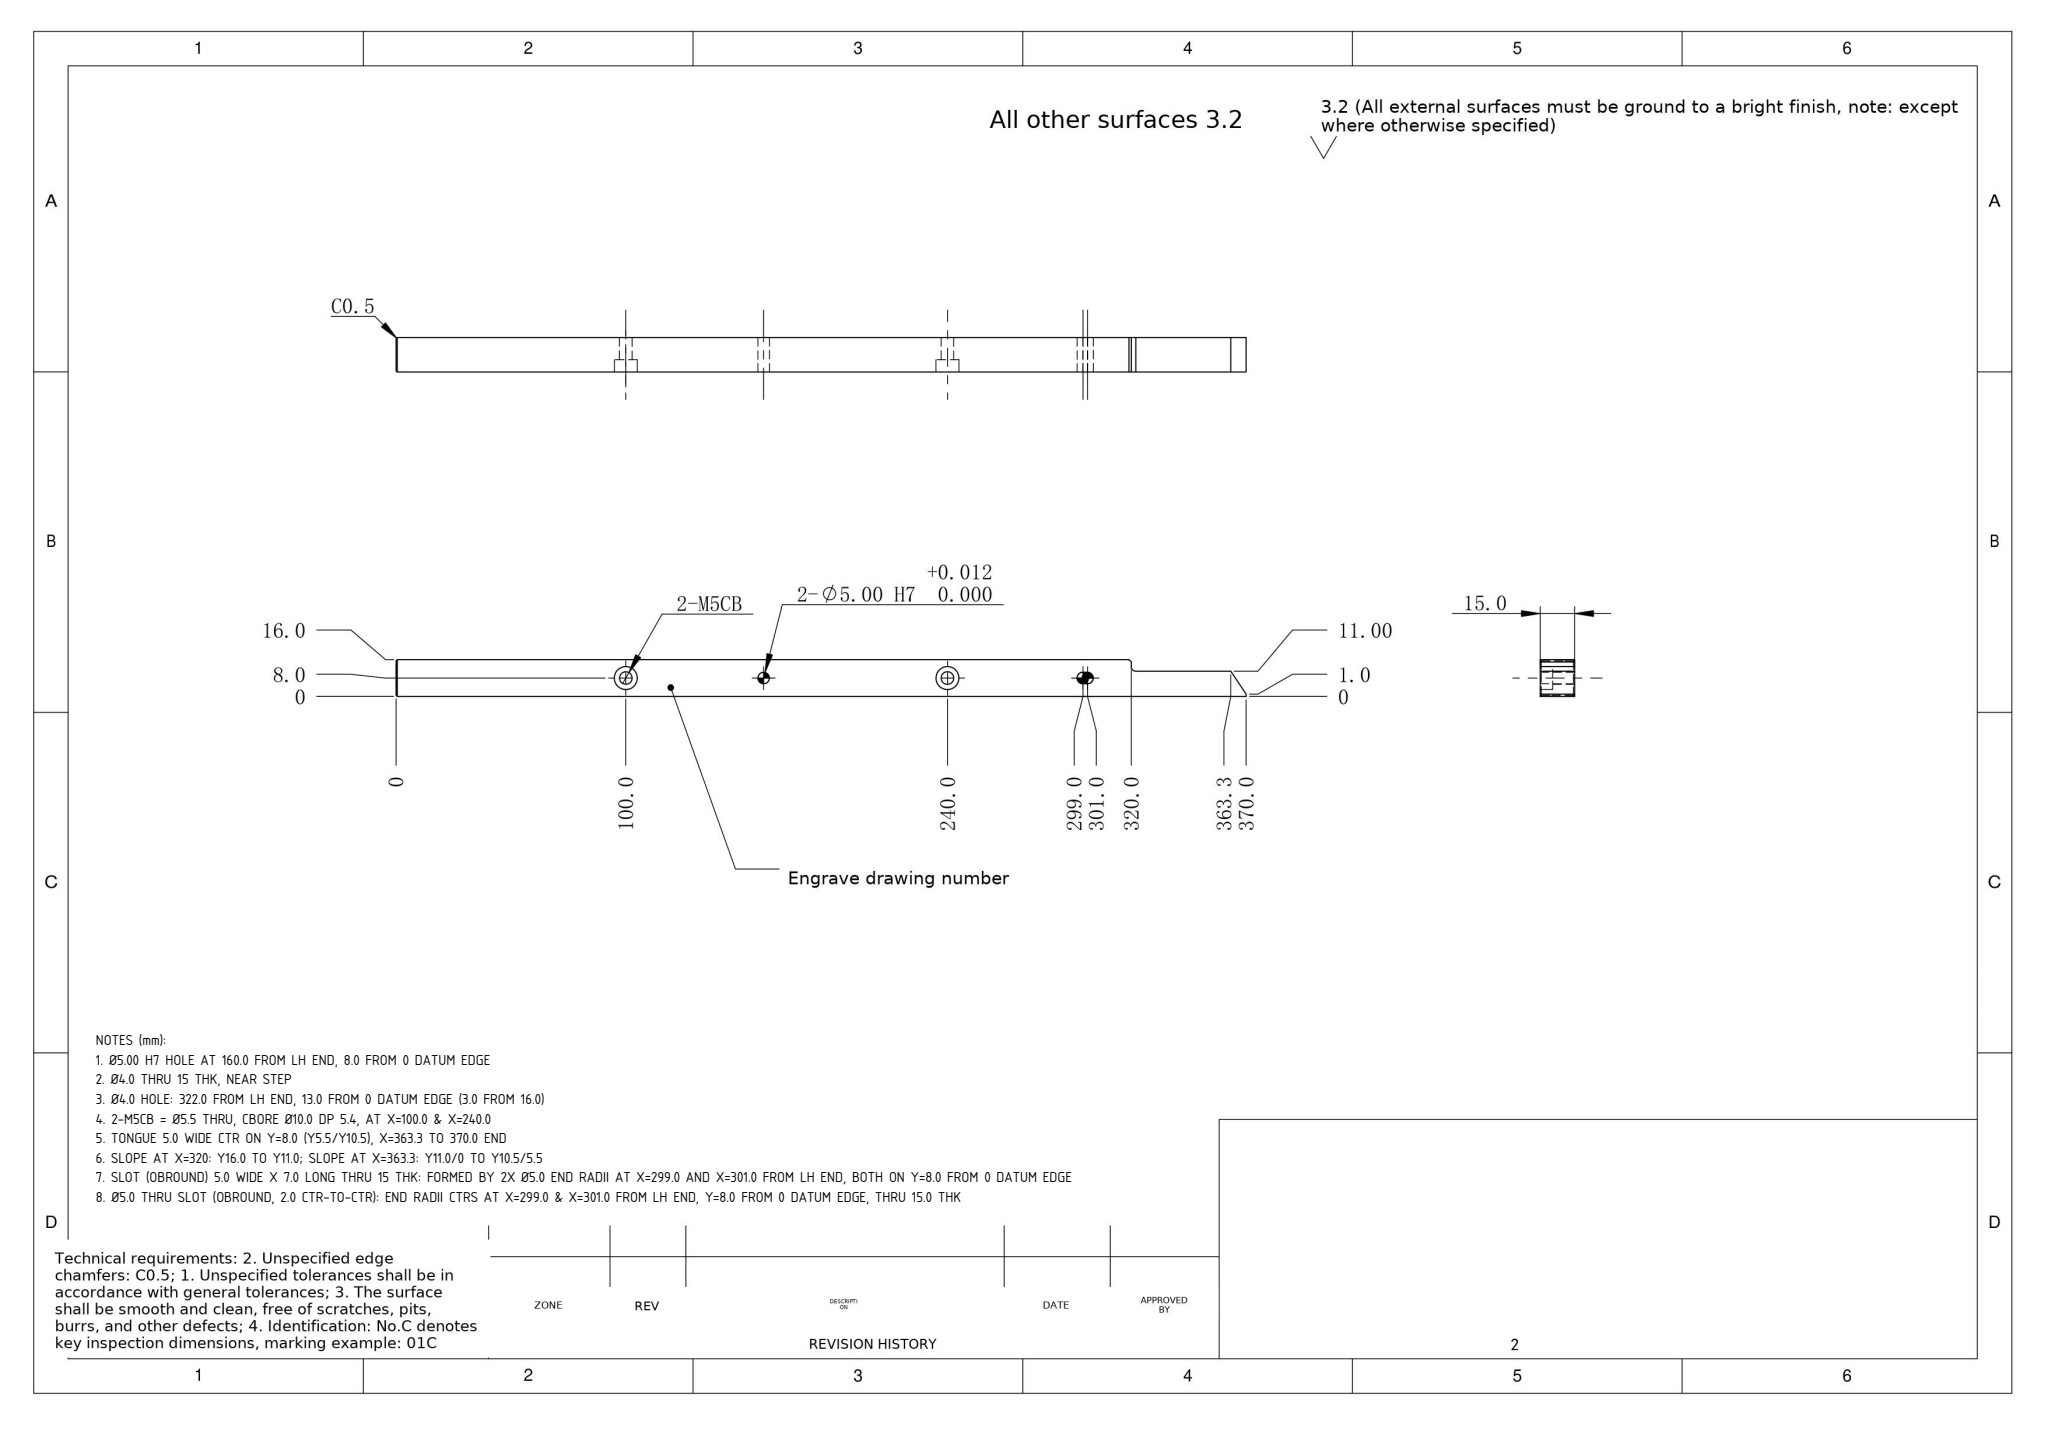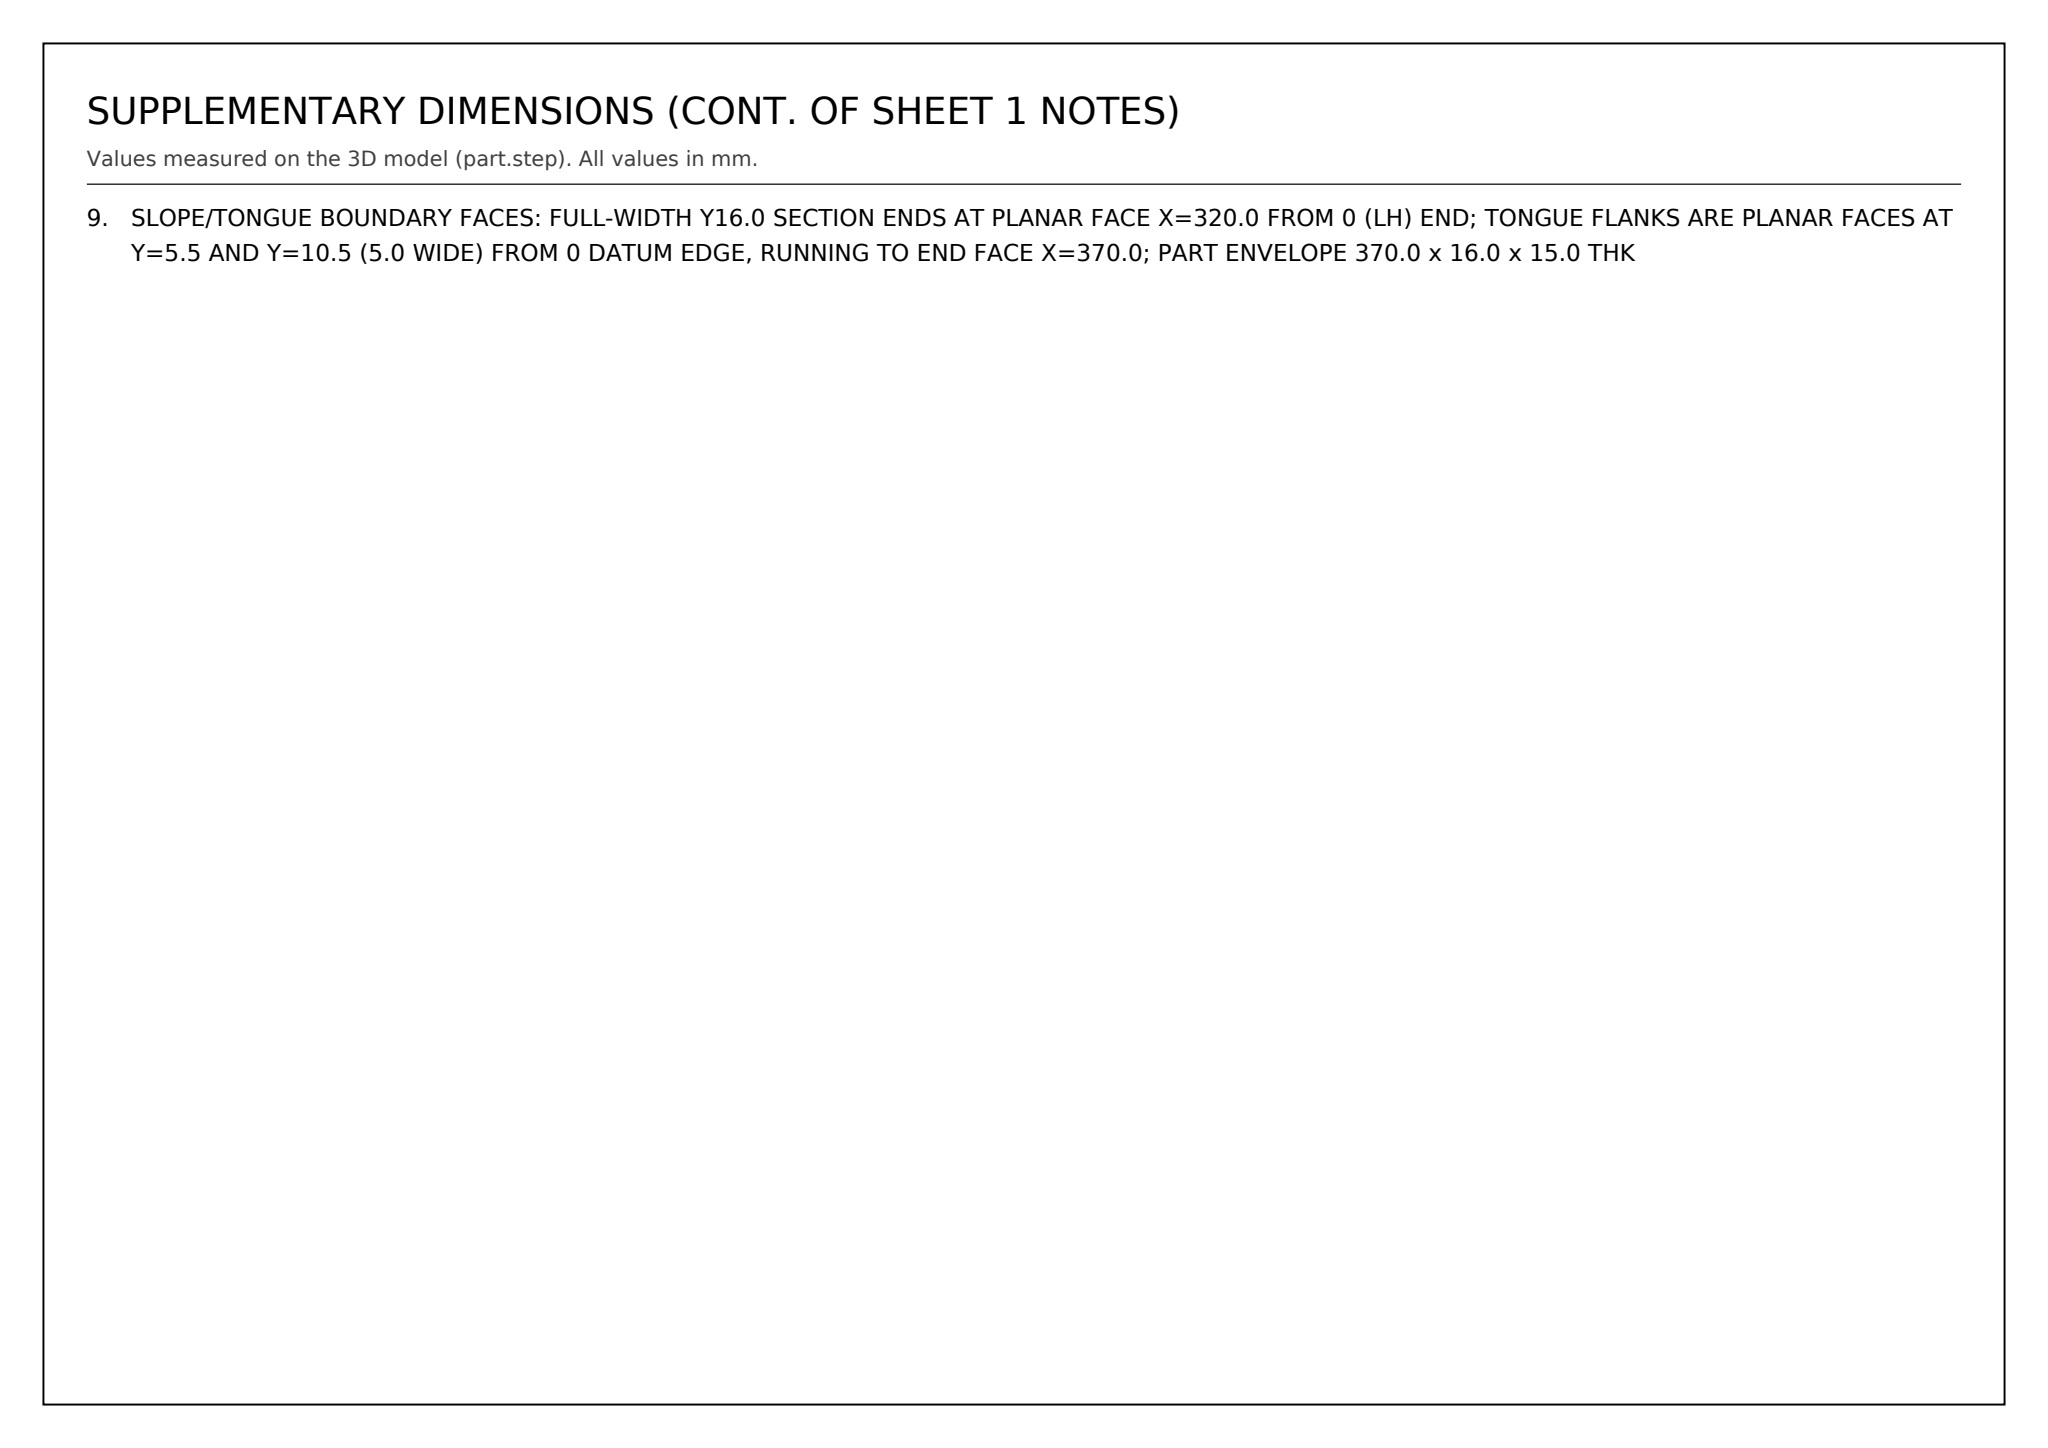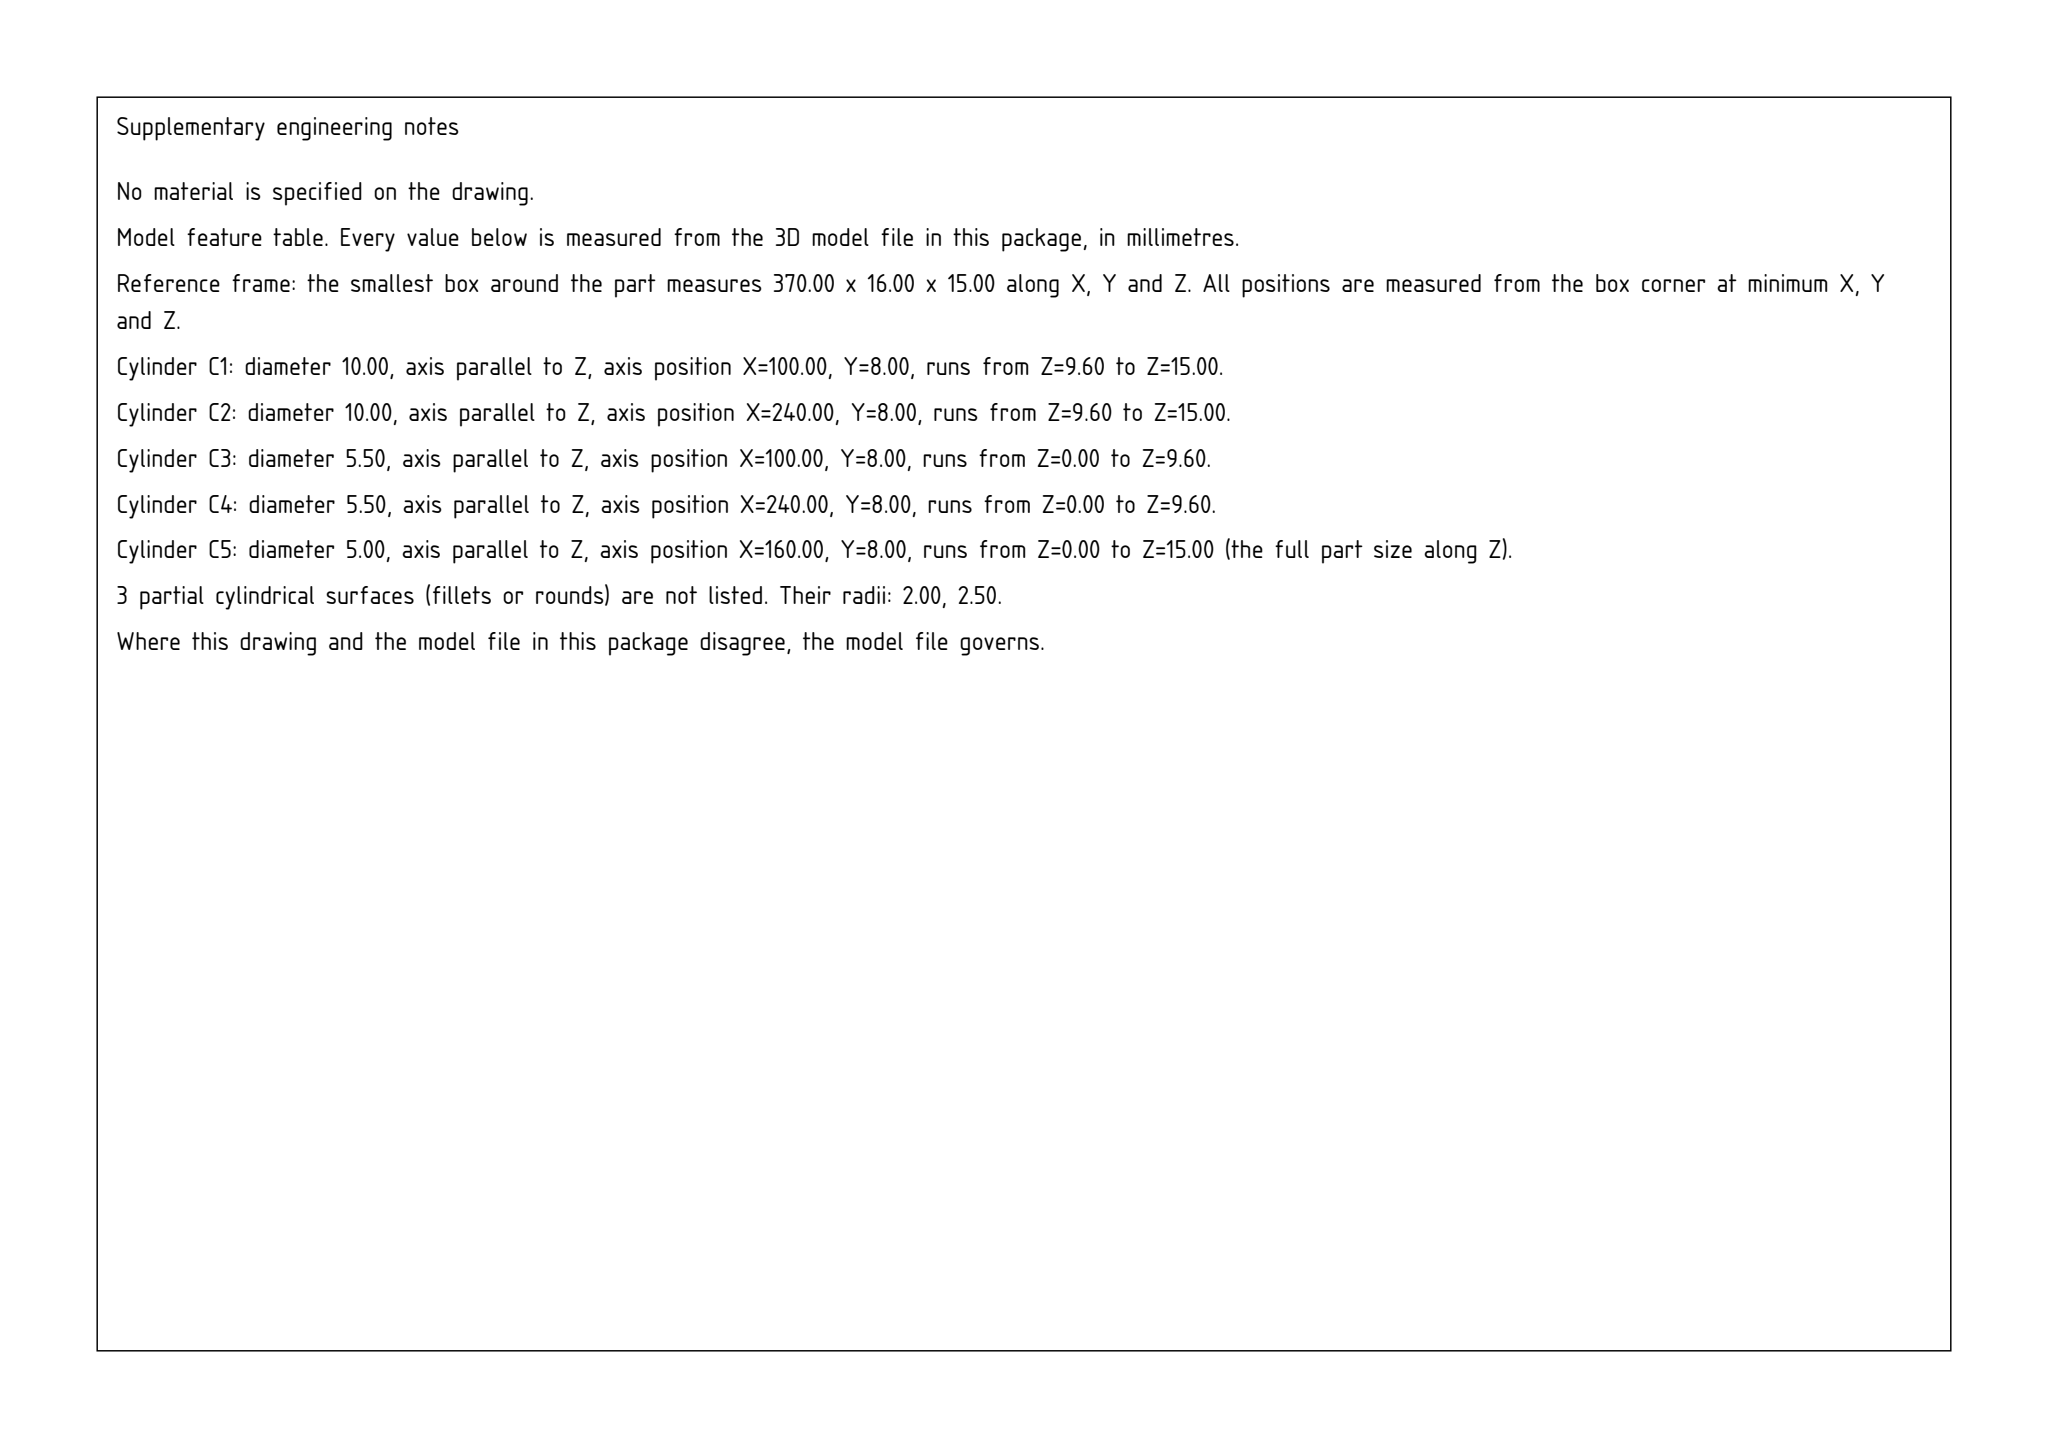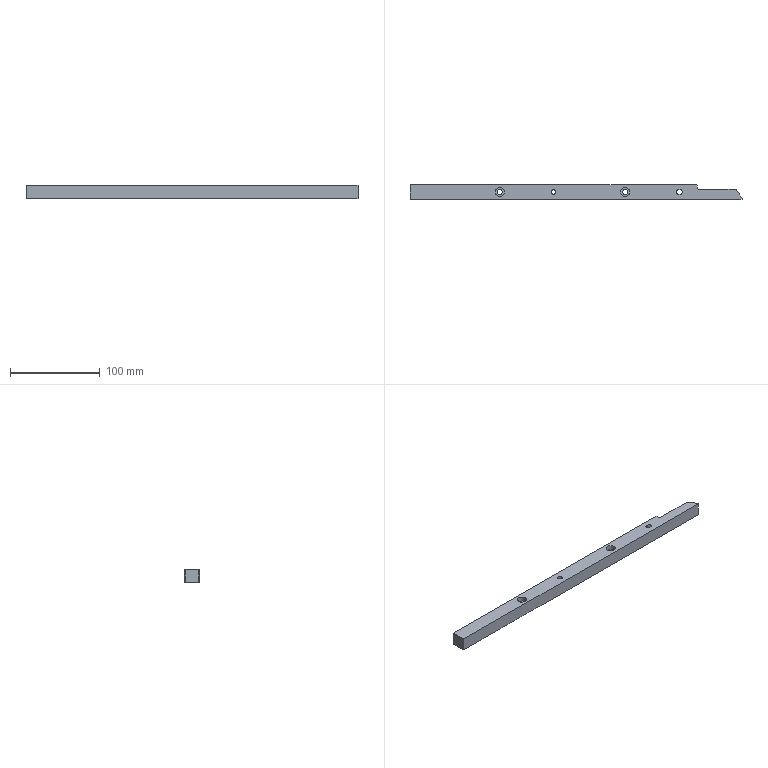Part | SolidWorks | mm | 1 solid | 32 faces | box 370 x 16 x 15 mm | volume 82504 mm3 | plane 18 | cylinder 14 | commonest cylinder face diameters 5 x5 10 x4 5.5 x4 4 x1
Drawing notes:
Ø5.00 H7 HOLE AT 160.0 FROM LH END, 8.0 FROM 0 DATUM EDGE | from the solid: cyl dia 5.0 axis z at (160.0, 8.0), len 15.0 (thru)
Ø4.0 THRU 15 THK, NEAR STEP | from the solid: cyl dia 4.0 axis z at (322.0, 13.0), len 15.0 = part thickness
Ø4.0 HOLE: 322.0 FROM LH END, 13.0 FROM 0 DATUM EDGE (3.0 FROM 16.0) | from the solid: cyl dia 4.0 pos x=322.0, y=13.0; y planes 0.0 and 16.0
2-M5CB = Ø5.5 THRU, CBORE Ø10.0 DP 5.4, AT X=100.0 & X=240.0 | from the solid: cyl Ø5.5 z @ (100,8) & (240,8) L9.6 thru; cyl Ø10.0 z same pos L5.4
TONGUE 5.0 WIDE CTR ON Y=8.0 (Y5.5/Y10.5), X=363.3 TO 370.0 END | from the solid: y-planes at 5.5 and 10.5; x-planes 370.0 end, 363.3 sloped face in view
SLOPE AT X=320: Y16.0 TO Y11.0; SLOPE AT X=363.3: Y11.0/0 TO Y10.5/5.5 | from the solid: y-planes 0,5.5,10.5,11.0,16.0; x-planes 0,320.0,370.0; no cones/fillets
SLOT (OBROUND) 5.0 WIDE X 7.0 LONG THRU 15 THK: FORMED BY 2X Ø5.0 END RADII AT X=299.0 AND X=301.0 FROM LH END, BOTH ON Y=8.0 FROM 0 DATUM EDGE | from the solid: cylinders: [5.0,'z',[299.0,8.0],15.0] and [5.0,'z',[301.0,8.0],15.0]; bbox z = 15.0
Ø5.0 THRU SLOT (OBROUND, 2.0 CTR-TO-CTR): END RADII CTRS AT X=299.0 & X=301.0 FROM LH END, Y=8.0 FROM 0 DATUM EDGE, THRU 15.0 THK | from the solid: cylinders: [5.0,'z',[299.0,8.0],15.0] and [5.0,'z',[301.0,8.0],15.0]; bbox_xyz z=15.0
SLOPE/TONGUE BOUNDARY FACES: FULL-WIDTH Y16.0 SECTION ENDS AT PLANAR FACE X=320.0 FROM 0 (LH) END; TONGUE FLANKS ARE PLANAR FACES AT Y=5.5 AND Y=10.5 (5.0 WIDE) FROM 0 DATUM EDGE, RUNNING TO END FACE X=370.0; PART ENVELOPE 370.0 x 16.0 x 15.0 THK | from the solid: axis_planes[x,0.0], [x,320.0], [x,370.0], [y,5.5], [y,10.5], [y,16.0], [z,0.0], [z,15.0]; bbox_xyz [370.0,16.0,15.0]
build123d program:
from build123d import *

# Parameters (mm, degrees)
SKETCH1_W                                       = 370
SKETCH1_H                                       = 16
BOSS_EXTRUDE1_DEPTH                             = 15
M5_HEX_SOCKET_HEAD_CAP_SCREW_CBORE1_D           = 5.5
M5_HEX_SOCKET_HEAD_CAP_SCREW_CBORE1_CBORE_D     = 10
M5_HEX_SOCKET_HEAD_CAP_SCREW_CBORE1_CBORE_DEPTH = 5.4
LPATTERN1_COUNT                                 = 2
LPATTERN1_PITCH                                 = 140
CHAMFER1_SIZE                                   = 15
CHAMFER1_SIZE2                                  = 10
CHAMFER2_SIZE                                   = 0.5
SKETCH4_R                                       = 2.5
CUT_EXTRUDE1_DEPTH                              = 371.649
SKETCH5_W                                       = 50
SKETCH5_H                                       = 5
CUT_EXTRUDE2_DEPTH                              = 371.649
CHAMFER3_SIZE                                   = 1
FILLET1_R                                       = 2


with BuildPart() as part:
    # Sketch1 → Boss-Extrude1 (new body)
    with BuildSketch(Plane.XY):
        with Locations((185, 8)):
            Rectangle(SKETCH1_W, SKETCH1_H)
    extrude(amount=BOSS_EXTRUDE1_DEPTH)

    # M5 Hex Socket Head Cap Screw CBORE1 (through all)
    with Locations(Plane.XY.offset(15)):
        with Locations((100, 8)):
            m5_hex_socket_head_cap_screw_cbore1 = CounterBoreHole(M5_HEX_SOCKET_HEAD_CAP_SCREW_CBORE1_D / 2, M5_HEX_SOCKET_HEAD_CAP_SCREW_CBORE1_CBORE_D / 2, M5_HEX_SOCKET_HEAD_CAP_SCREW_CBORE1_CBORE_DEPTH)

    # LPattern1: M5 Hex Socket Head Cap Screw CBORE1 ×2
    with Locations(*[(i * LPATTERN1_PITCH, 0, 0) for i in range(1, LPATTERN1_COUNT)]):
        add(m5_hex_socket_head_cap_screw_cbore1, mode=Mode.SUBTRACT)

    # Chamfer1
    chamfer1_edges = [part.edges().sort_by_distance(p)[0] for p in [
        (370, 16, 7.5),
    ]]
    chamfer1_side = [part.faces().sort_by_distance(p)[0] for p in [
        (370, 8, 7.5),
    ]]
    chamfer(chamfer1_edges, length=CHAMFER1_SIZE, length2=CHAMFER1_SIZE2, reference=chamfer1_side[0])

    # Chamfer2
    chamfer2_edges = [part.edges().sort_by_distance(p)[0] for p in [
        (0, 8, 15),
        (0, 8, 0),
        (0, 16, 7.5),
        (0, 0, 7.5),
    ]]
    chamfer(chamfer2_edges, length=CHAMFER2_SIZE)

    # Sketch4 → Cut-Extrude1 (cut, through all)
    with BuildSketch(Plane.XY.offset(15)):
        with Locations((160, 8)):
            Circle(SKETCH4_R)
        with BuildLine():
            Line((301, 5.5), (299, 5.5))
            ThreePointArc((299, 5.5), (296.5, 8), (299, 10.5))
            Line((299, 10.5), (301, 10.5))
            ThreePointArc((301, 10.5), (303.5, 8), (301, 5.5))
        make_face()
    extrude(amount=-CUT_EXTRUDE1_DEPTH, mode=Mode.SUBTRACT)

    # Sketch5 → Cut-Extrude2 (cut, through all)
    with BuildSketch(Plane.XY.offset(15)):
        with Locations((345, 13.5)):
            Rectangle(SKETCH5_W, SKETCH5_H)
    extrude(amount=-CUT_EXTRUDE2_DEPTH, mode=Mode.SUBTRACT)

    # Chamfer3
    chamfer3_edges = [part.edges().sort_by_distance(p)[0] for p in [
        (320, 16, 7.5),
    ]]
    chamfer(chamfer3_edges, length=CHAMFER3_SIZE)

    # Fillet1
    fillet1_edges = [part.edges().sort_by_distance(p)[0] for p in [
        (320, 11, 7.5),
    ]]
    fillet(fillet1_edges, radius=FILLET1_R)


solid = part.part